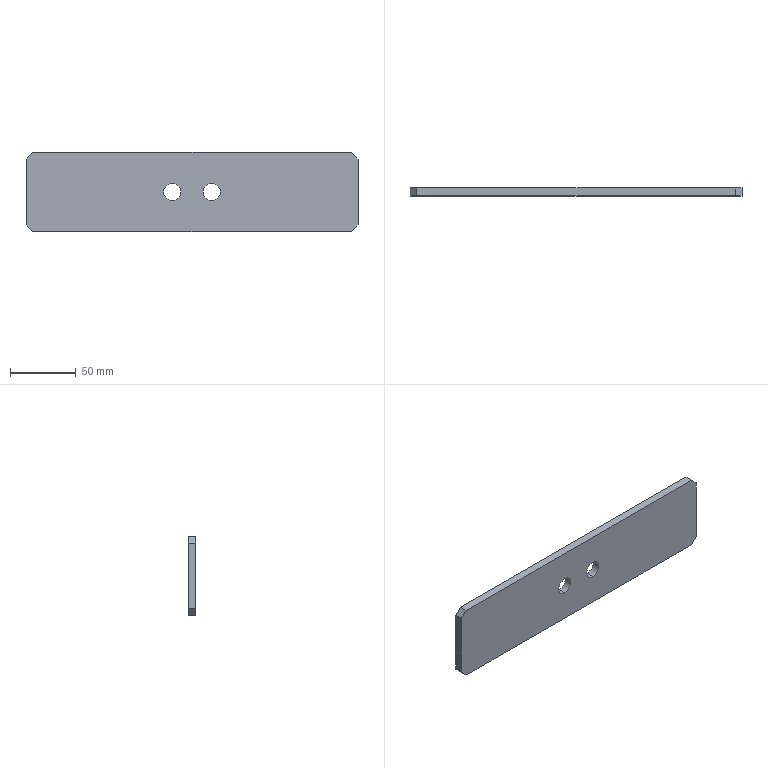Component | SolidWorks | THK-B1011LooseRopeProtectionMountingPlate-1 | 1 solid | 14 faces | box 252 x 6 x 60 mm | volume 88827 mm3 | plane 10 | cylinder 4 | commonest cylinder face diameters 13 x4 | material Q235A
build123d program:
from build123d import *

# Parameters (mm, degrees)
SKETCH1_W                  = 252
SKETCH1_H                  = 60
BOSS_EXTRUDE1_DEPTH        = 3
F_13_0_13_DIAMETER_HOLE1_D = 13
CHAMFER1_SIZE              = 5


with BuildPart() as part:
    # Sketch1 → Boss-Extrude1 (new, symmetric)
    with BuildSketch(Plane(origin=(0, 0, 0), x_dir=(1, 0, 0), z_dir=(0, 1, 0))):
        Rectangle(SKETCH1_W, SKETCH1_H)
    extrude(amount=BOSS_EXTRUDE1_DEPTH, both=True)

    # 13.0 _13_ Diameter Hole1 (through all)
    with Locations(Plane(origin=(0, 3, 0), x_dir=(1, 0, 0), z_dir=(0, 1, 0))):
        with Locations((-15, 0), (15, 0)):
            Hole(F_13_0_13_DIAMETER_HOLE1_D / 2)

    # Chamfer1
    chamfer1_edges = [part.edges().sort_by_distance(p)[0] for p in [
        (126, 0, 30),
        (-126, 0, 30),
        (-126, 0, -30),
        (126, 0, -30),
    ]]
    chamfer(chamfer1_edges, length=CHAMFER1_SIZE)


solid = part.part

# Placed as in the assembly
solid = solid.moved(Location((0, 23, -225), (0, 0, 0)))
STEP:
#1=CARTESIAN_POINT('',(-0.5906,0.7874,-9.114));
#2=VERTEX_POINT('',#1);
#3=CARTESIAN_POINT('',(-0.5906,0.7874,-8.602));
#4=VERTEX_POINT('',#3);
#5=CARTESIAN_POINT('',(-0.5906,0.7874,-8.858));
#6=DIRECTION('',(0.,1.,0.));
#7=DIRECTION('',(0.,0.,1.));
#8=AXIS2_PLACEMENT_3D('',#5,#6,#7);
#9=CIRCLE('',#8,0.2559);
#10=EDGE_CURVE('',#2,#4,#9,.T.);
#11=ORIENTED_EDGE('',*,*,#10,.F.);
#12=CARTESIAN_POINT('',(-0.5906,1.024,-9.114));
#13=VERTEX_POINT('',#12);
#14=CARTESIAN_POINT('',(-0.5906,1.024,-9.114));
#15=DIRECTION('',(0.,1.,0.));
#16=VECTOR('',#15,39.37);
#17=LINE('',#14,#16);
#18=EDGE_CURVE('',#2,#13,#17,.T.);
#19=ORIENTED_EDGE('',*,*,#18,.T.);
#20=CARTESIAN_POINT('',(-0.5906,1.024,-8.602));
#21=VERTEX_POINT('',#20);
#22=CARTESIAN_POINT('',(-0.5906,1.024,-8.858));
#23=DIRECTION('',(0.,1.,0.));
#24=DIRECTION('',(0.,0.,1.));
#25=AXIS2_PLACEMENT_3D('',#22,#23,#24);
#26=CIRCLE('',#25,0.2559);
#27=EDGE_CURVE('',#13,#21,#26,.T.);
#28=ORIENTED_EDGE('',*,*,#27,.T.);
#29=CARTESIAN_POINT('',(-0.5906,1.024,-8.602));
#30=DIRECTION('',(0.,1.,0.));
#31=VECTOR('',#30,39.37);
#32=LINE('',#29,#31);
#33=EDGE_CURVE('',#4,#21,#32,.T.);
#34=ORIENTED_EDGE('',*,*,#33,.F.);
#35=EDGE_LOOP('',(#11,#19,#28,#34));
#36=FACE_OUTER_BOUND('',#35,.T.);
#37=CARTESIAN_POINT('',(-0.5906,1.024,-8.858));
#38=DIRECTION('',(0.,1.,0.));
#39=DIRECTION('',(0.,0.,1.));
#40=AXIS2_PLACEMENT_3D('',#37,#38,#39);
#41=CYLINDRICAL_SURFACE('',#40,0.2559);
#42=ADVANCED_FACE('',(#36),#41,.F.);
#43=CARTESIAN_POINT('',(0.5906,0.7874,-9.114));
#44=VERTEX_POINT('',#43);
#45=CARTESIAN_POINT('',(0.5906,0.7874,-8.602));
#46=VERTEX_POINT('',#45);
#47=CARTESIAN_POINT('',(0.5906,0.7874,-8.858));
#48=DIRECTION('',(0.,1.,0.));
#49=DIRECTION('',(0.,0.,1.));
#50=AXIS2_PLACEMENT_3D('',#47,#48,#49);
#51=CIRCLE('',#50,0.2559);
#52=EDGE_CURVE('',#44,#46,#51,.T.);
#53=ORIENTED_EDGE('',*,*,#52,.F.);
#54=CARTESIAN_POINT('',(0.5906,1.024,-9.114));
#55=VERTEX_POINT('',#54);
#56=CARTESIAN_POINT('',(0.5906,1.024,-9.114));
#57=DIRECTION('',(0.,1.,0.));
#58=VECTOR('',#57,39.37);
#59=LINE('',#56,#58);
#60=EDGE_CURVE('',#44,#55,#59,.T.);
#61=ORIENTED_EDGE('',*,*,#60,.T.);
#62=CARTESIAN_POINT('',(0.5906,1.024,-8.602));
#63=VERTEX_POINT('',#62);
#64=CARTESIAN_POINT('',(0.5906,1.024,-8.858));
#65=DIRECTION('',(0.,1.,0.));
#66=DIRECTION('',(0.,0.,1.));
#67=AXIS2_PLACEMENT_3D('',#64,#65,#66);
#68=CIRCLE('',#67,0.2559);
#69=EDGE_CURVE('',#55,#63,#68,.T.);
#70=ORIENTED_EDGE('',*,*,#69,.T.);
#71=CARTESIAN_POINT('',(0.5906,1.024,-8.602));
#72=DIRECTION('',(0.,1.,0.));
#73=VECTOR('',#72,39.37);
#74=LINE('',#71,#73);
#75=EDGE_CURVE('',#46,#63,#74,.T.);
#76=ORIENTED_EDGE('',*,*,#75,.F.);
#77=EDGE_LOOP('',(#53,#61,#70,#76));
#78=FACE_OUTER_BOUND('',#77,.T.);
#79=CARTESIAN_POINT('',(0.5906,1.024,-8.858));
#80=DIRECTION('',(0.,1.,0.));
#81=DIRECTION('',(0.,0.,1.));
#82=AXIS2_PLACEMENT_3D('',#79,#80,#81);
#83=CYLINDRICAL_SURFACE('',#82,0.2559);
#84=ADVANCED_FACE('',(#78),#83,.F.);
#85=CARTESIAN_POINT('',(4.961,1.024,-7.874));
#86=VERTEX_POINT('',#85);
#87=CARTESIAN_POINT('',(4.961,1.024,-9.843));
#88=VERTEX_POINT('',#87);
#89=CARTESIAN_POINT('',(4.961,1.024,-7.677));
#90=DIRECTION('',(0.,0.,-1.));
#91=VECTOR('',#90,39.37);
#92=LINE('',#89,#91);
#93=EDGE_CURVE('',#86,#88,#92,.T.);
#94=ORIENTED_EDGE('',*,*,#93,.F.);
#95=CARTESIAN_POINT('',(4.961,0.7874,-7.874));
#96=VERTEX_POINT('',#95);
#97=CARTESIAN_POINT('',(4.961,1.024,-7.874));
#98=DIRECTION('',(0.,-1.,0.));
#99=VECTOR('',#98,39.37);
#100=LINE('',#97,#99);
#101=EDGE_CURVE('',#86,#96,#100,.T.);
#102=ORIENTED_EDGE('',*,*,#101,.T.);
#103=CARTESIAN_POINT('',(4.961,0.7874,-9.843));
#104=VERTEX_POINT('',#103);
#105=CARTESIAN_POINT('',(4.961,0.7874,-7.677));
#106=DIRECTION('',(0.,0.,-1.));
#107=VECTOR('',#106,39.37);
#108=LINE('',#105,#107);
#109=EDGE_CURVE('',#96,#104,#108,.T.);
#110=ORIENTED_EDGE('',*,*,#109,.T.);
#111=CARTESIAN_POINT('',(4.961,1.024,-9.843));
#112=DIRECTION('',(0.,1.,0.));
#113=VECTOR('',#112,39.37);
#114=LINE('',#111,#113);
#115=EDGE_CURVE('',#104,#88,#114,.T.);
#116=ORIENTED_EDGE('',*,*,#115,.T.);
#117=EDGE_LOOP('',(#94,#102,#110,#116));
#118=FACE_OUTER_BOUND('',#117,.T.);
#119=CARTESIAN_POINT('',(4.961,1.024,-7.677));
#120=DIRECTION('',(-1.,0.,0.));
#121=DIRECTION('',(0.,0.,1.));
#122=AXIS2_PLACEMENT_3D('',#119,#120,#121);
#123=PLANE('',#122);
#124=ADVANCED_FACE('',(#118),#123,.F.);
#125=CARTESIAN_POINT('',(4.764,0.7874,-10.039));
#126=VERTEX_POINT('',#125);
#127=CARTESIAN_POINT('',(-4.764,0.7874,-10.039));
#128=VERTEX_POINT('',#127);
#129=CARTESIAN_POINT('',(-4.961,0.7874,-10.039));
#130=DIRECTION('',(-1.,0.,0.));
#131=VECTOR('',#130,39.37);
#132=LINE('',#129,#131);
#133=EDGE_CURVE('',#126,#128,#132,.T.);
#134=ORIENTED_EDGE('',*,*,#133,.T.);
#135=CARTESIAN_POINT('',(-4.764,1.024,-10.039));
#136=VERTEX_POINT('',#135);
#137=CARTESIAN_POINT('',(-4.764,1.024,-10.039));
#138=DIRECTION('',(0.,1.,0.));
#139=VECTOR('',#138,39.37);
#140=LINE('',#137,#139);
#141=EDGE_CURVE('',#128,#136,#140,.T.);
#142=ORIENTED_EDGE('',*,*,#141,.T.);
#143=CARTESIAN_POINT('',(4.764,1.024,-10.039));
#144=VERTEX_POINT('',#143);
#145=CARTESIAN_POINT('',(-4.961,1.024,-10.039));
#146=DIRECTION('',(-1.,0.,0.));
#147=VECTOR('',#146,39.37);
#148=LINE('',#145,#147);
#149=EDGE_CURVE('',#144,#136,#148,.T.);
#150=ORIENTED_EDGE('',*,*,#149,.F.);
#151=CARTESIAN_POINT('',(4.764,1.024,-10.039));
#152=DIRECTION('',(0.,-1.,0.));
#153=VECTOR('',#152,39.37);
#154=LINE('',#151,#153);
#155=EDGE_CURVE('',#144,#126,#154,.T.);
#156=ORIENTED_EDGE('',*,*,#155,.T.);
#157=EDGE_LOOP('',(#134,#142,#150,#156));
#158=FACE_OUTER_BOUND('',#157,.T.);
#159=CARTESIAN_POINT('',(-4.961,1.024,-10.039));
#160=DIRECTION('',(0.,0.,1.));
#161=DIRECTION('',(1.,0.,0.));
#162=AXIS2_PLACEMENT_3D('',#159,#160,#161);
#163=PLANE('',#162);
#164=ADVANCED_FACE('',(#158),#163,.F.);
#165=CARTESIAN_POINT('',(-4.961,0.7874,-9.843));
#166=VERTEX_POINT('',#165);
#167=CARTESIAN_POINT('',(-4.961,0.7874,-7.874));
#168=VERTEX_POINT('',#167);
#169=CARTESIAN_POINT('',(-4.961,0.7874,-7.677));
#170=DIRECTION('',(0.,0.,1.));
#171=VECTOR('',#170,39.37);
#172=LINE('',#169,#171);
#173=EDGE_CURVE('',#166,#168,#172,.T.);
#174=ORIENTED_EDGE('',*,*,#173,.T.);
#175=CARTESIAN_POINT('',(-4.961,1.024,-7.874));
#176=VERTEX_POINT('',#175);
#177=CARTESIAN_POINT('',(-4.961,1.024,-7.874));
#178=DIRECTION('',(0.,1.,0.));
#179=VECTOR('',#178,39.37);
#180=LINE('',#177,#179);
#181=EDGE_CURVE('',#168,#176,#180,.T.);
#182=ORIENTED_EDGE('',*,*,#181,.T.);
#183=CARTESIAN_POINT('',(-4.961,1.024,-9.843));
#184=VERTEX_POINT('',#183);
#185=CARTESIAN_POINT('',(-4.961,1.024,-7.677));
#186=DIRECTION('',(0.,0.,1.));
#187=VECTOR('',#186,39.37);
#188=LINE('',#185,#187);
#189=EDGE_CURVE('',#184,#176,#188,.T.);
#190=ORIENTED_EDGE('',*,*,#189,.F.);
#191=CARTESIAN_POINT('',(-4.961,1.024,-9.843));
#192=DIRECTION('',(0.,-1.,0.));
#193=VECTOR('',#192,39.37);
#194=LINE('',#191,#193);
#195=EDGE_CURVE('',#184,#166,#194,.T.);
#196=ORIENTED_EDGE('',*,*,#195,.T.);
#197=EDGE_LOOP('',(#174,#182,#190,#196));
#198=FACE_OUTER_BOUND('',#197,.T.);
#199=CARTESIAN_POINT('',(-4.961,1.024,-7.677));
#200=DIRECTION('',(1.,0.,0.));
#201=DIRECTION('',(0.,0.,-1.));
#202=AXIS2_PLACEMENT_3D('',#199,#200,#201);
#203=PLANE('',#202);
#204=ADVANCED_FACE('',(#198),#203,.F.);
#205=CARTESIAN_POINT('',(-4.764,1.024,-7.677));
#206=VERTEX_POINT('',#205);
#207=CARTESIAN_POINT('',(4.764,1.024,-7.677));
#208=VERTEX_POINT('',#207);
#209=CARTESIAN_POINT('',(-4.961,1.024,-7.677));
#210=DIRECTION('',(1.,0.,0.));
#211=VECTOR('',#210,39.37);
#212=LINE('',#209,#211);
#213=EDGE_CURVE('',#206,#208,#212,.T.);
#214=ORIENTED_EDGE('',*,*,#213,.F.);
#215=CARTESIAN_POINT('',(-4.764,0.7874,-7.677));
#216=VERTEX_POINT('',#215);
#217=CARTESIAN_POINT('',(-4.764,1.024,-7.677));
#218=DIRECTION('',(0.,-1.,0.));
#219=VECTOR('',#218,39.37);
#220=LINE('',#217,#219);
#221=EDGE_CURVE('',#206,#216,#220,.T.);
#222=ORIENTED_EDGE('',*,*,#221,.T.);
#223=CARTESIAN_POINT('',(4.764,0.7874,-7.677));
#224=VERTEX_POINT('',#223);
#225=CARTESIAN_POINT('',(-4.961,0.7874,-7.677));
#226=DIRECTION('',(1.,0.,0.));
#227=VECTOR('',#226,39.37);
#228=LINE('',#225,#227);
#229=EDGE_CURVE('',#216,#224,#228,.T.);
#230=ORIENTED_EDGE('',*,*,#229,.T.);
#231=CARTESIAN_POINT('',(4.764,1.024,-7.677));
#232=DIRECTION('',(0.,1.,0.));
#233=VECTOR('',#232,39.37);
#234=LINE('',#231,#233);
#235=EDGE_CURVE('',#224,#208,#234,.T.);
#236=ORIENTED_EDGE('',*,*,#235,.T.);
#237=EDGE_LOOP('',(#214,#222,#230,#236));
#238=FACE_OUTER_BOUND('',#237,.T.);
#239=CARTESIAN_POINT('',(-4.961,1.024,-7.677));
#240=DIRECTION('',(0.,0.,-1.));
#241=DIRECTION('',(-1.,0.,0.));
#242=AXIS2_PLACEMENT_3D('',#239,#240,#241);
#243=PLANE('',#242);
#244=ADVANCED_FACE('',(#238),#243,.F.);
#245=CARTESIAN_POINT('',(-0.5906,1.024,-8.858));
#246=DIRECTION('',(0.,1.,0.));
#247=DIRECTION('',(0.,0.,1.));
#248=AXIS2_PLACEMENT_3D('',#245,#246,#247);
#249=CIRCLE('',#248,0.2559);
#250=EDGE_CURVE('',#21,#13,#249,.T.);
#251=ORIENTED_EDGE('',*,*,#250,.F.);
#252=ORIENTED_EDGE('',*,*,#27,.F.);
#253=EDGE_LOOP('',(#251,#252));
#254=FACE_BOUND('',#253,.T.);
#255=CARTESIAN_POINT('',(0.5906,1.024,-8.858));
#256=DIRECTION('',(0.,1.,0.));
#257=DIRECTION('',(0.,0.,1.));
#258=AXIS2_PLACEMENT_3D('',#255,#256,#257);
#259=CIRCLE('',#258,0.2559);
#260=EDGE_CURVE('',#63,#55,#259,.T.);
#261=ORIENTED_EDGE('',*,*,#260,.F.);
#262=ORIENTED_EDGE('',*,*,#69,.F.);
#263=EDGE_LOOP('',(#261,#262));
#264=FACE_BOUND('',#263,.T.);
#265=ORIENTED_EDGE('',*,*,#189,.T.);
#266=CARTESIAN_POINT('',(-4.764,1.024,-7.677));
#267=DIRECTION('',(0.7071,0.,0.7071));
#268=VECTOR('',#267,39.37);
#269=LINE('',#266,#268);
#270=EDGE_CURVE('',#176,#206,#269,.T.);
#271=ORIENTED_EDGE('',*,*,#270,.T.);
#272=ORIENTED_EDGE('',*,*,#213,.T.);
#273=CARTESIAN_POINT('',(4.961,1.024,-7.874));
#274=DIRECTION('',(0.7071,0.,-0.7071));
#275=VECTOR('',#274,39.37);
#276=LINE('',#273,#275);
#277=EDGE_CURVE('',#208,#86,#276,.T.);
#278=ORIENTED_EDGE('',*,*,#277,.T.);
#279=ORIENTED_EDGE('',*,*,#93,.T.);
#280=CARTESIAN_POINT('',(4.764,1.024,-10.039));
#281=DIRECTION('',(-0.7071,0.,-0.7071));
#282=VECTOR('',#281,39.37);
#283=LINE('',#280,#282);
#284=EDGE_CURVE('',#88,#144,#283,.T.);
#285=ORIENTED_EDGE('',*,*,#284,.T.);
#286=ORIENTED_EDGE('',*,*,#149,.T.);
#287=CARTESIAN_POINT('',(-4.961,1.024,-9.843));
#288=DIRECTION('',(-0.7071,0.,0.7071));
#289=VECTOR('',#288,39.37);
#290=LINE('',#287,#289);
#291=EDGE_CURVE('',#136,#184,#290,.T.);
#292=ORIENTED_EDGE('',*,*,#291,.T.);
#293=EDGE_LOOP('',(#265,#271,#272,#278,#279,#285,#286,#292));
#294=FACE_OUTER_BOUND('',#293,.T.);
#295=CARTESIAN_POINT('',(0.,1.024,-8.858));
#296=DIRECTION('',(0.,-1.,0.));
#297=DIRECTION('',(0.,0.,-1.));
#298=AXIS2_PLACEMENT_3D('',#295,#296,#297);
#299=PLANE('',#298);
#300=ADVANCED_FACE('',(#254,#264,#294),#299,.F.);
#301=CARTESIAN_POINT('',(-0.5906,0.7874,-8.858));
#302=DIRECTION('',(0.,1.,0.));
#303=DIRECTION('',(0.,0.,1.));
#304=AXIS2_PLACEMENT_3D('',#301,#302,#303);
#305=CIRCLE('',#304,0.2559);
#306=EDGE_CURVE('',#4,#2,#305,.T.);
#307=ORIENTED_EDGE('',*,*,#306,.T.);
#308=ORIENTED_EDGE('',*,*,#10,.T.);
#309=EDGE_LOOP('',(#307,#308));
#310=FACE_BOUND('',#309,.T.);
#311=CARTESIAN_POINT('',(0.5906,0.7874,-8.858));
#312=DIRECTION('',(0.,1.,0.));
#313=DIRECTION('',(0.,0.,1.));
#314=AXIS2_PLACEMENT_3D('',#311,#312,#313);
#315=CIRCLE('',#314,0.2559);
#316=EDGE_CURVE('',#46,#44,#315,.T.);
#317=ORIENTED_EDGE('',*,*,#316,.T.);
#318=ORIENTED_EDGE('',*,*,#52,.T.);
#319=EDGE_LOOP('',(#317,#318));
#320=FACE_BOUND('',#319,.T.);
#321=ORIENTED_EDGE('',*,*,#229,.F.);
#322=CARTESIAN_POINT('',(-2.972,0.7874,-5.886));
#323=DIRECTION('',(-0.7071,0.,-0.7071));
#324=VECTOR('',#323,39.37);
#325=LINE('',#322,#324);
#326=EDGE_CURVE('',#216,#168,#325,.T.);
#327=ORIENTED_EDGE('',*,*,#326,.T.);
#328=ORIENTED_EDGE('',*,*,#173,.F.);
#329=CARTESIAN_POINT('',(-2.972,0.7874,-11.831));
#330=DIRECTION('',(0.7071,0.,-0.7071));
#331=VECTOR('',#330,39.37);
#332=LINE('',#329,#331);
#333=EDGE_CURVE('',#166,#128,#332,.T.);
#334=ORIENTED_EDGE('',*,*,#333,.T.);
#335=ORIENTED_EDGE('',*,*,#133,.F.);
#336=CARTESIAN_POINT('',(2.972,0.7874,-11.831));
#337=DIRECTION('',(0.7071,0.,0.7071));
#338=VECTOR('',#337,39.37);
#339=LINE('',#336,#338);
#340=EDGE_CURVE('',#126,#104,#339,.T.);
#341=ORIENTED_EDGE('',*,*,#340,.T.);
#342=ORIENTED_EDGE('',*,*,#109,.F.);
#343=CARTESIAN_POINT('',(2.972,0.7874,-5.886));
#344=DIRECTION('',(-0.7071,0.,0.7071));
#345=VECTOR('',#344,39.37);
#346=LINE('',#343,#345);
#347=EDGE_CURVE('',#96,#224,#346,.T.);
#348=ORIENTED_EDGE('',*,*,#347,.T.);
#349=EDGE_LOOP('',(#321,#327,#328,#334,#335,#341,#342,#348));
#350=FACE_OUTER_BOUND('',#349,.T.);
#351=CARTESIAN_POINT('',(0.,0.7874,-8.858));
#352=DIRECTION('',(0.,-1.,0.));
#353=DIRECTION('',(0.,0.,-1.));
#354=AXIS2_PLACEMENT_3D('',#351,#352,#353);
#355=PLANE('',#354);
#356=ADVANCED_FACE('',(#310,#320,#350),#355,.T.);
#357=ORIENTED_EDGE('',*,*,#60,.F.);
#358=ORIENTED_EDGE('',*,*,#316,.F.);
#359=ORIENTED_EDGE('',*,*,#75,.T.);
#360=ORIENTED_EDGE('',*,*,#260,.T.);
#361=EDGE_LOOP('',(#357,#358,#359,#360));
#362=FACE_OUTER_BOUND('',#361,.T.);
#363=CARTESIAN_POINT('',(0.5906,1.024,-8.858));
#364=DIRECTION('',(0.,1.,0.));
#365=DIRECTION('',(0.,0.,1.));
#366=AXIS2_PLACEMENT_3D('',#363,#364,#365);
#367=CYLINDRICAL_SURFACE('',#366,0.2559);
#368=ADVANCED_FACE('',(#362),#367,.F.);
#369=ORIENTED_EDGE('',*,*,#18,.F.);
#370=ORIENTED_EDGE('',*,*,#306,.F.);
#371=ORIENTED_EDGE('',*,*,#33,.T.);
#372=ORIENTED_EDGE('',*,*,#250,.T.);
#373=EDGE_LOOP('',(#369,#370,#371,#372));
#374=FACE_OUTER_BOUND('',#373,.T.);
#375=CARTESIAN_POINT('',(-0.5906,1.024,-8.858));
#376=DIRECTION('',(0.,1.,0.));
#377=DIRECTION('',(0.,0.,1.));
#378=AXIS2_PLACEMENT_3D('',#375,#376,#377);
#379=CYLINDRICAL_SURFACE('',#378,0.2559);
#380=ADVANCED_FACE('',(#374),#379,.F.);
#381=ORIENTED_EDGE('',*,*,#270,.F.);
#382=ORIENTED_EDGE('',*,*,#181,.F.);
#383=ORIENTED_EDGE('',*,*,#326,.F.);
#384=ORIENTED_EDGE('',*,*,#221,.F.);
#385=EDGE_LOOP('',(#381,#382,#383,#384));
#386=FACE_OUTER_BOUND('',#385,.T.);
#387=CARTESIAN_POINT('',(-4.764,1.024,-7.677));
#388=DIRECTION('',(0.7071,0.,-0.7071));
#389=DIRECTION('',(0.,-1.,0.));
#390=AXIS2_PLACEMENT_3D('',#387,#388,#389);
#391=PLANE('',#390);
#392=ADVANCED_FACE('',(#386),#391,.F.);
#393=ORIENTED_EDGE('',*,*,#291,.F.);
#394=ORIENTED_EDGE('',*,*,#141,.F.);
#395=ORIENTED_EDGE('',*,*,#333,.F.);
#396=ORIENTED_EDGE('',*,*,#195,.F.);
#397=EDGE_LOOP('',(#393,#394,#395,#396));
#398=FACE_OUTER_BOUND('',#397,.T.);
#399=CARTESIAN_POINT('',(-4.961,1.024,-9.843));
#400=DIRECTION('',(0.7071,0.,0.7071));
#401=DIRECTION('',(0.,-1.,0.));
#402=AXIS2_PLACEMENT_3D('',#399,#400,#401);
#403=PLANE('',#402);
#404=ADVANCED_FACE('',(#398),#403,.F.);
#405=ORIENTED_EDGE('',*,*,#277,.F.);
#406=ORIENTED_EDGE('',*,*,#235,.F.);
#407=ORIENTED_EDGE('',*,*,#347,.F.);
#408=ORIENTED_EDGE('',*,*,#101,.F.);
#409=EDGE_LOOP('',(#405,#406,#407,#408));
#410=FACE_OUTER_BOUND('',#409,.T.);
#411=CARTESIAN_POINT('',(4.961,1.024,-7.874));
#412=DIRECTION('',(-0.7071,0.,-0.7071));
#413=DIRECTION('',(0.,-1.,0.));
#414=AXIS2_PLACEMENT_3D('',#411,#412,#413);
#415=PLANE('',#414);
#416=ADVANCED_FACE('',(#410),#415,.F.);
#417=ORIENTED_EDGE('',*,*,#284,.F.);
#418=ORIENTED_EDGE('',*,*,#115,.F.);
#419=ORIENTED_EDGE('',*,*,#340,.F.);
#420=ORIENTED_EDGE('',*,*,#155,.F.);
#421=EDGE_LOOP('',(#417,#418,#419,#420));
#422=FACE_OUTER_BOUND('',#421,.T.);
#423=CARTESIAN_POINT('',(4.764,1.024,-10.039));
#424=DIRECTION('',(-0.7071,0.,0.7071));
#425=DIRECTION('',(0.,-1.,0.));
#426=AXIS2_PLACEMENT_3D('',#423,#424,#425);
#427=PLANE('',#426);
#428=ADVANCED_FACE('',(#422),#427,.F.);
#429=CLOSED_SHELL('',(#42,#84,#124,#164,#204,#244,#300,#356,#368,#380,#392,#404,#416,#428));
#430=MANIFOLD_SOLID_BREP('',#429);
#431=CARTESIAN_POINT('',(0.,0.,0.));
#432=DIRECTION('',(0.,0.,1.));
#433=DIRECTION('',(1.,0.,0.));
#434=AXIS2_PLACEMENT_3D('',#431,#432,#433);
#435=(LENGTH_UNIT()NAMED_UNIT(*)SI_UNIT($,.METRE.));
#436=LENGTH_MEASURE_WITH_UNIT(LENGTH_MEASURE(0.0254),#435);
#437=DIMENSIONAL_EXPONENTS(1.,0.,0.,0.,0.,0.,0.);
#438=(CONVERSION_BASED_UNIT('',#436)LENGTH_UNIT()NAMED_UNIT(#437));
#439=UNCERTAINTY_MEASURE_WITH_UNIT(LENGTH_MEASURE(0.00001),#438,'','');
#440=(NAMED_UNIT(*)PLANE_ANGLE_UNIT()SI_UNIT($,.RADIAN.));
#441=(NAMED_UNIT(*)SI_UNIT($,.STERADIAN.)SOLID_ANGLE_UNIT());
#442=(GEOMETRIC_REPRESENTATION_CONTEXT(3)GLOBAL_UNCERTAINTY_ASSIGNED_CONTEXT((#439))GLOBAL_UNIT_ASSIGNED_CONTEXT((#438,#440,#441))REPRESENTATION_CONTEXT('',''));
#443=ADVANCED_BREP_SHAPE_REPRESENTATION('',(#430,#434),#442);
#444=COLOUR_RGB('',0.7922,0.8196,0.9333);
#445=FILL_AREA_STYLE_COLOUR('',#444);
#446=FILL_AREA_STYLE('',(#445));
#447=SURFACE_STYLE_FILL_AREA(#446);
#448=SURFACE_SIDE_STYLE('',(#447));
#449=SURFACE_STYLE_USAGE(.BOTH.,#448);
#450=PRESENTATION_STYLE_ASSIGNMENT((#449));
#451=STYLED_ITEM('',(#450),#430);
#452=PRESENTATION_LAYER_ASSIGNMENT('','',(#451));
#453=(LENGTH_UNIT()NAMED_UNIT(*)SI_UNIT($,.METRE.));
#454=LENGTH_MEASURE_WITH_UNIT(LENGTH_MEASURE(0.0254),#453);
#455=DIMENSIONAL_EXPONENTS(1.,0.,0.,0.,0.,0.,0.);
#456=(CONVERSION_BASED_UNIT('',#454)LENGTH_UNIT()NAMED_UNIT(#455));
#457=UNCERTAINTY_MEASURE_WITH_UNIT(LENGTH_MEASURE(0.00001),#456,'','');
#458=(NAMED_UNIT(*)PLANE_ANGLE_UNIT()SI_UNIT($,.RADIAN.));
#459=(NAMED_UNIT(*)SI_UNIT($,.STERADIAN.)SOLID_ANGLE_UNIT());
#460=(GEOMETRIC_REPRESENTATION_CONTEXT(3)GLOBAL_UNCERTAINTY_ASSIGNED_CONTEXT((#457))GLOBAL_UNIT_ASSIGNED_CONTEXT((#456,#458,#459))REPRESENTATION_CONTEXT('',''));
#461=MECHANICAL_DESIGN_GEOMETRIC_PRESENTATION_REPRESENTATION('',(#451),#460);